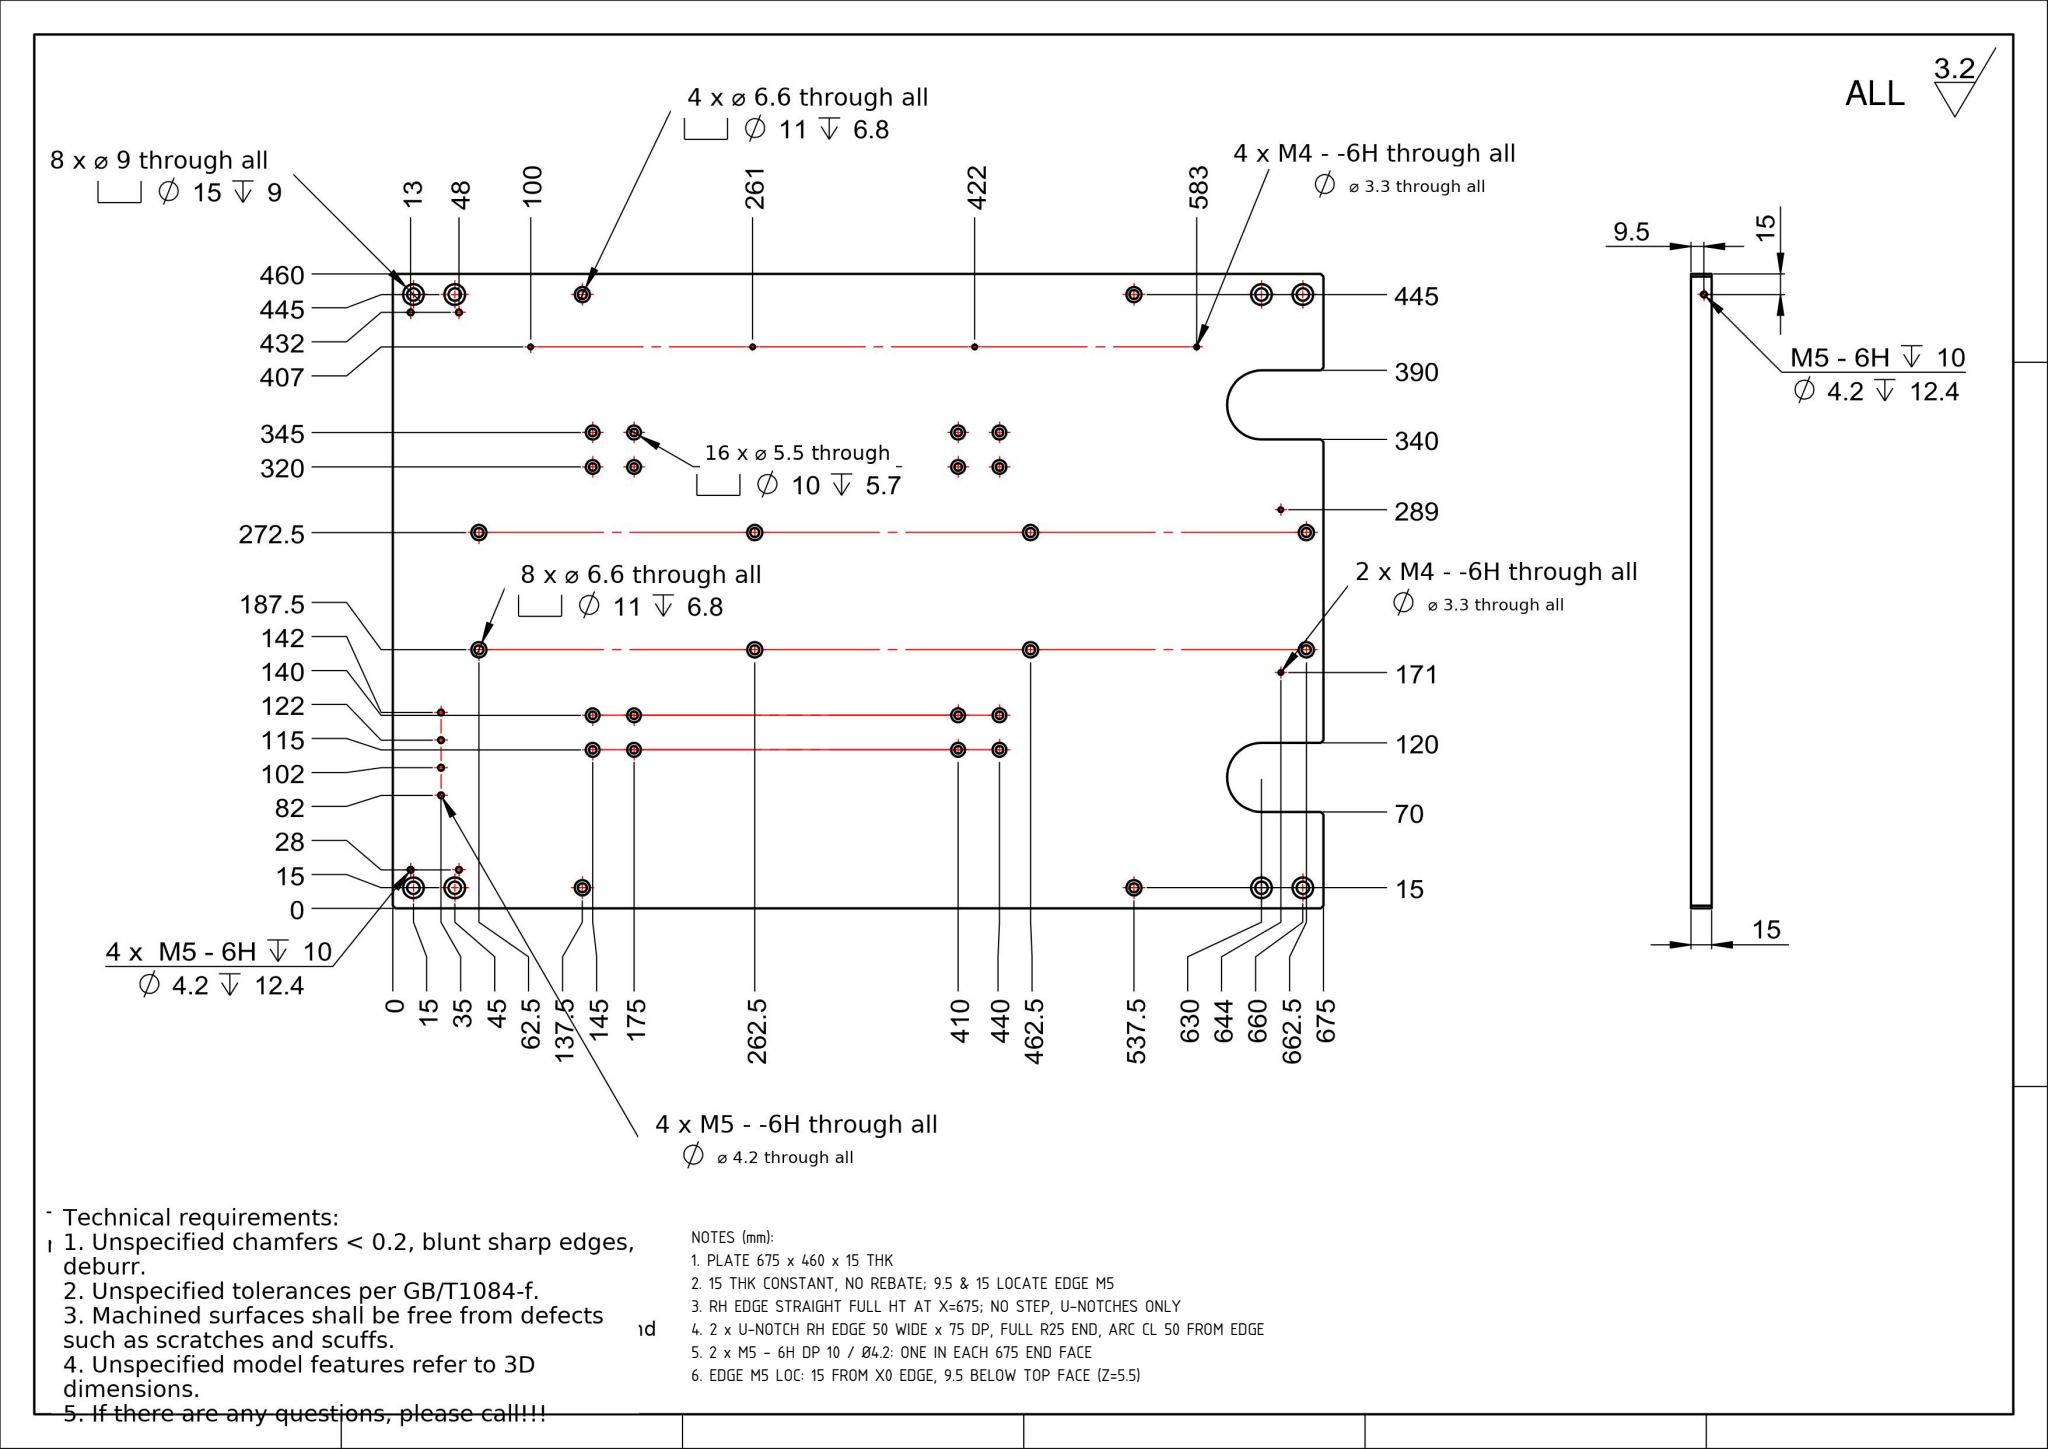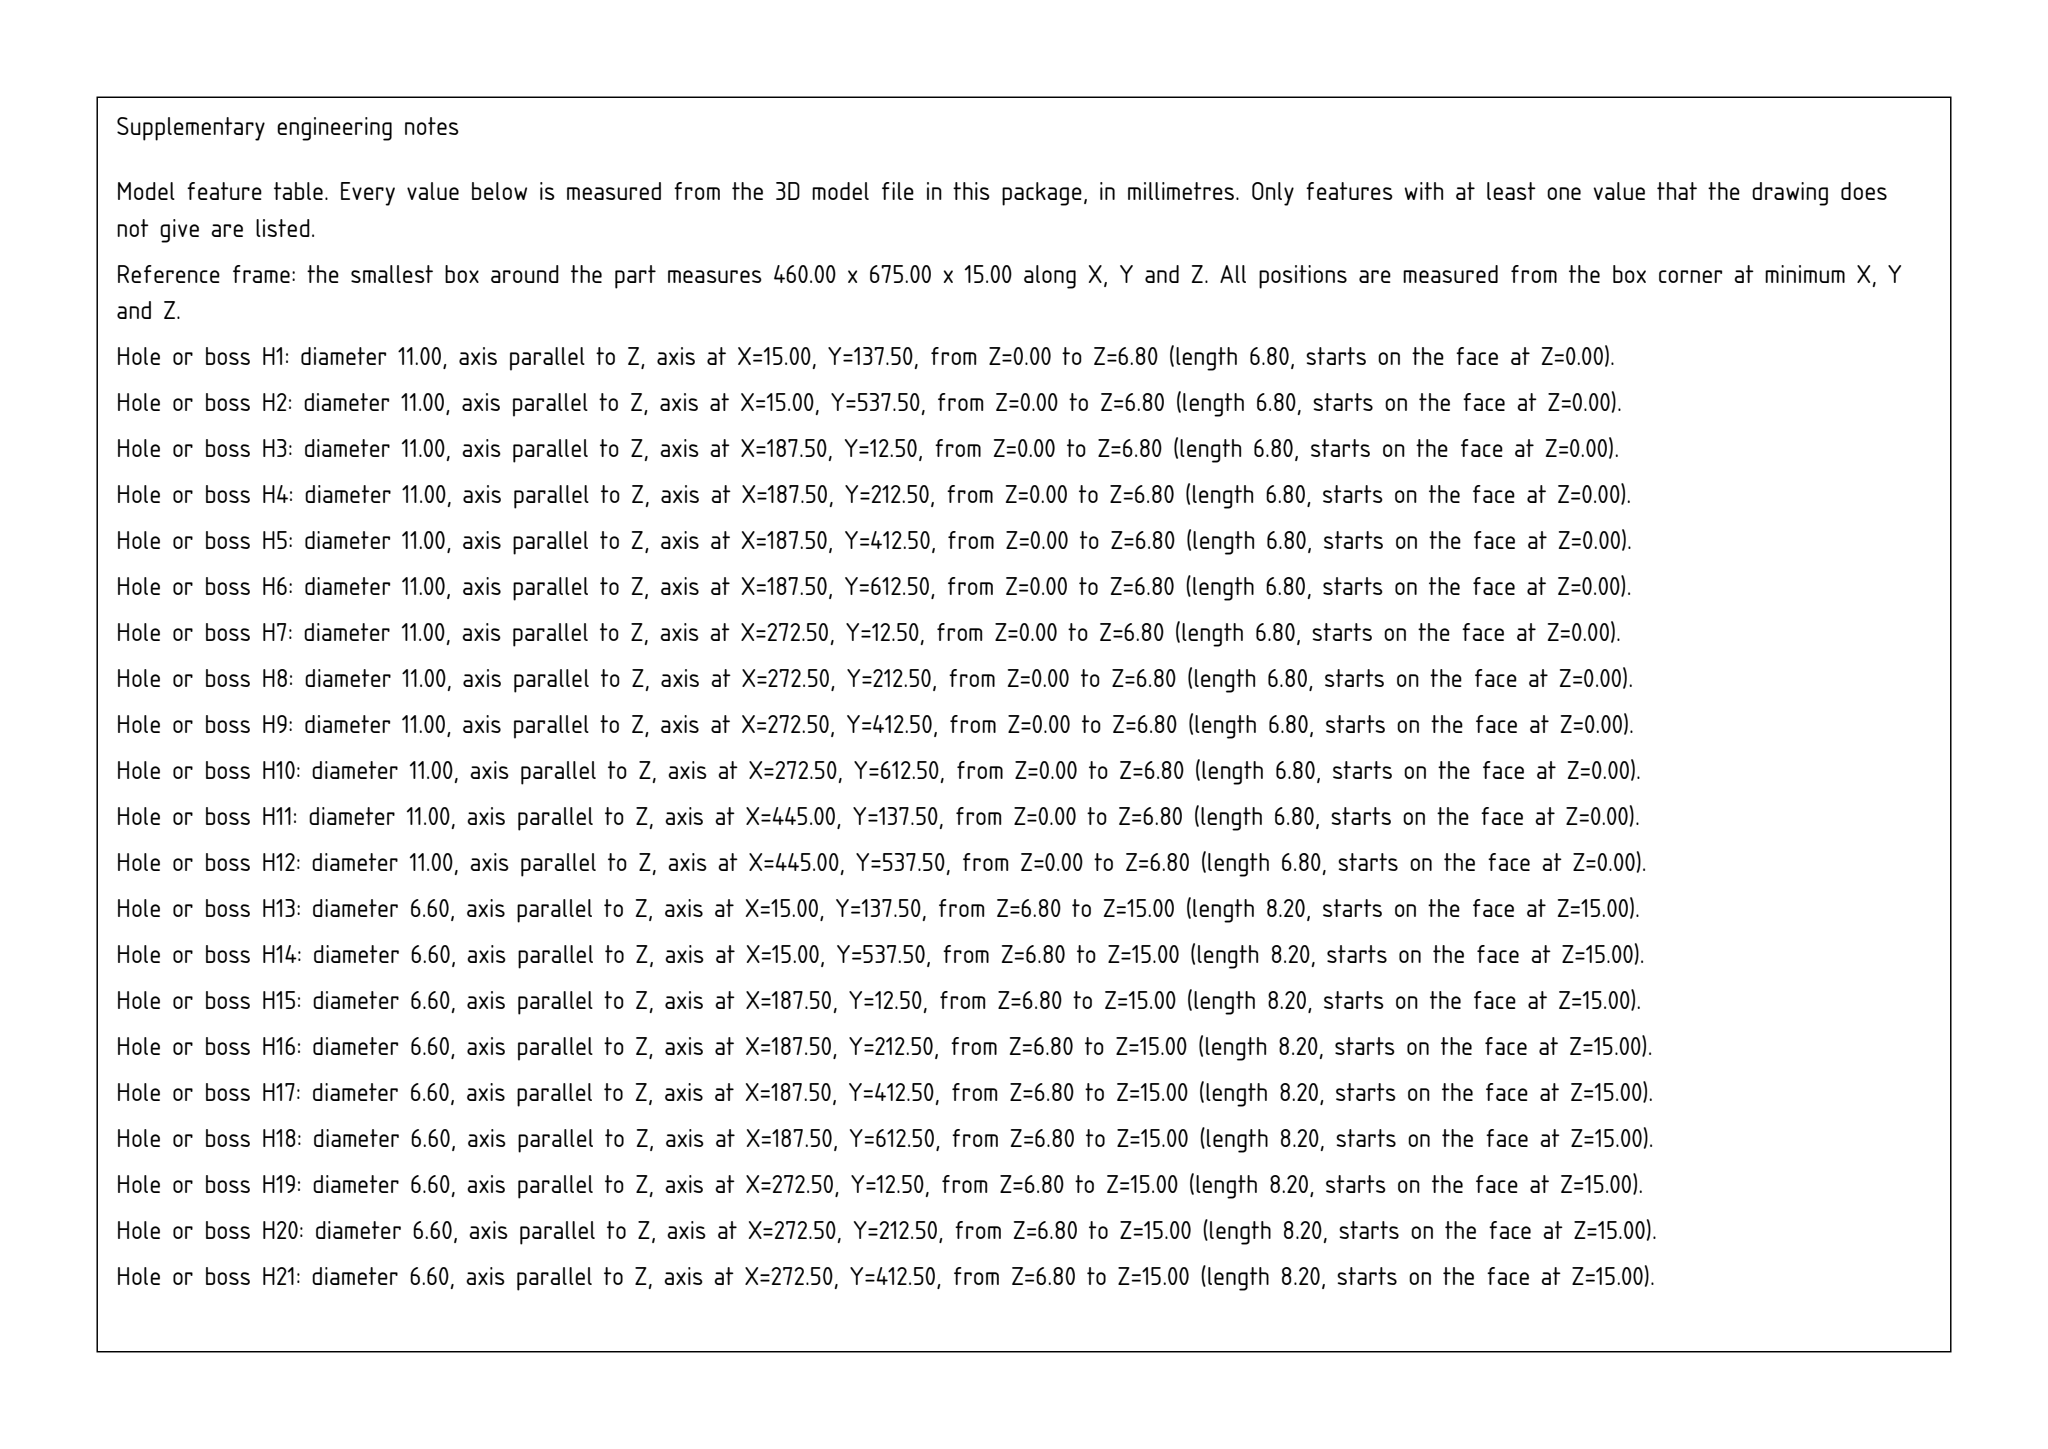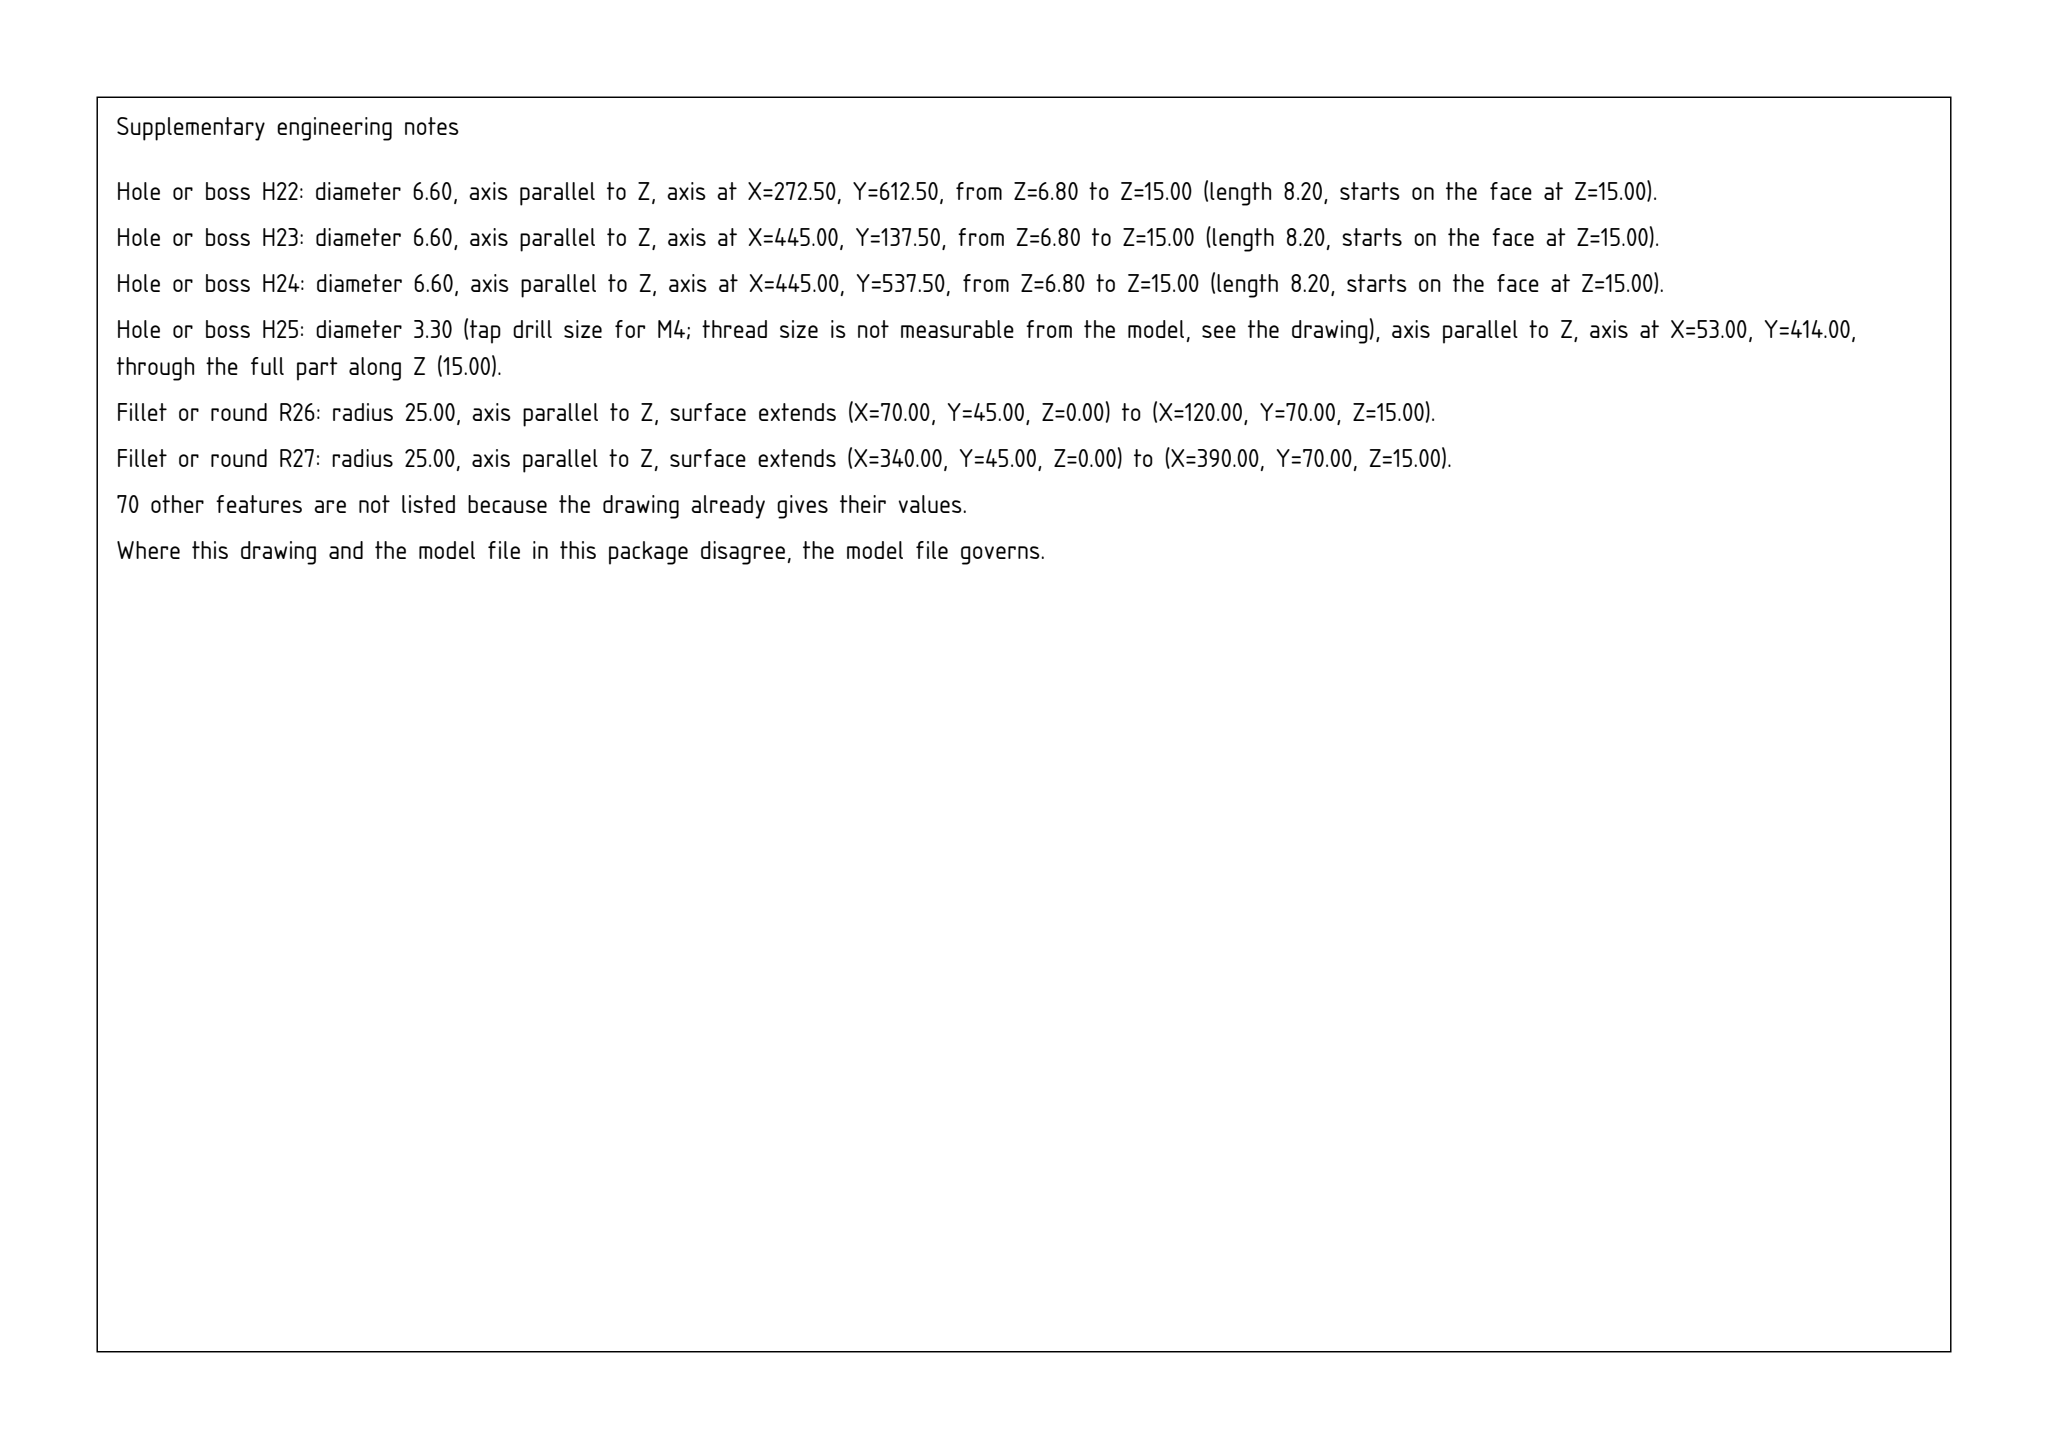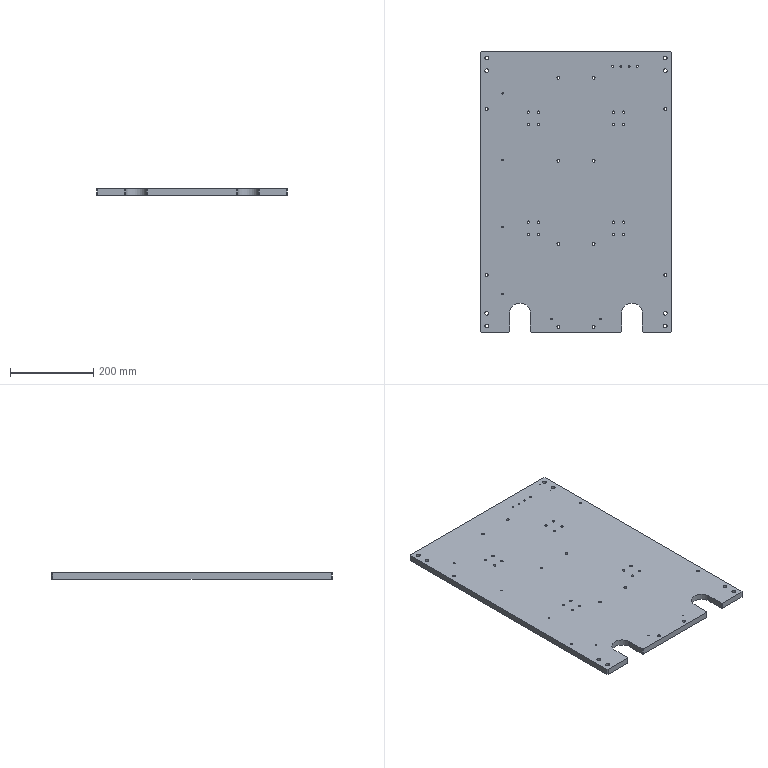Part | SolidWorks | mm | 1 solid | 240 faces | box 460 x 675 x 15 mm | volume 4520295 mm3 | cylinder 176 | plane 56 | cone 8 | commonest cylinder face diameters 10 x32 5.5 x32 11 x24 6.6 x24 4.2 x18 15 x16 9 x16 3.3 x12
Drawing notes:
PLATE 675 x 460 x 15 THK | from the solid: bbox_xyz [460,675,15]
15 THK CONSTANT, NO REBATE; 9.5 & 15 LOCATE EDGE M5 | from the solid: z-planes only 0.0 and 15.0 full faces = uniform plate; Ø4.2 y-axis hole at x=15, z=5.5 (9.5 below z=15 face)
RH EDGE STRAIGHT FULL HT AT X=675; NO STEP, U-NOTCHES ONLY | from the solid: axis_planes ['y',0.0] count 3 coplanar RH-edge faces (drawing X=675); only other y-plane is 675 (LH edge)
2 x U-NOTCH RH EDGE 50 WIDE x 75 DP, FULL R25 END, ARC CL 50 FROM EDGE | from the solid: notch flats x=70/120 and x=340/390 = 50 wide, running in from y=0 RH edge; full R25 end, arc centre 50 in = 75 total depth
2 x M5 - 6H DP 10 / Ø4.2: ONE IN EACH 675 END FACE | from the solid: cylinders [4.2,"y",[15.0,null,5.5],7.8, count 2] - axis along Y, one hole in each y-end face (y=0 and y=675) of 460x675x15 bbox
EDGE M5 LOC: 15 FROM X0 EDGE, 9.5 BELOW TOP FACE (Z=5.5) | from the solid: hole axis at x=15.0, z=5.5; thickness 15 so 15-5.5=9.5 from top face, matching 9.5 & 15 in side view
build123d program:
from build123d import *

# Parameters (mm, degrees)
SKETCH1_W                                         = 460
SKETCH1_H                                         = 675
BOSS_EXTRUDE1_DEPTH                               = 7.5
HOLE_SIZE_ACCORDING_TO_HEXAGON_SOCKET_D           = 6.6
HOLE_SIZE_ACCORDING_TO_HEXAGON_SOCKET_CBORE_D     = 11
HOLE_SIZE_ACCORDING_TO_HEXAGON_SOCKET_CBORE_DEPTH = 6.8
M8_HEX_SOCKET_HEAD_CAP_SCREW_CBORE3_D             = 9
M8_HEX_SOCKET_HEAD_CAP_SCREW_CBORE3_CBORE_D       = 15
M8_HEX_SOCKET_HEAD_CAP_SCREW_CBORE3_CBORE_DEPTH   = 9
M5_TAPPED_HOLE2_D                                 = 4.2
HOLE_SIZE_ACCORDING_TO_HEXAGON_SO_2_D             = 6.6
HOLE_SIZE_ACCORDING_TO_HEXAGON_SO_2_CBORE_D       = 11
HOLE_SIZE_ACCORDING_TO_HEXAGON_SO_2_CBORE_DEPTH   = 6.8
M4_TAPPED_HOLE3_D                                 = 3.3
LPATTERN3_COUNT                                   = 4
LPATTERN3_PITCH                                   = 161
HOLE_SIZE_ACCORDING_TO_HEXAGON_SO_3_D             = 5.5
HOLE_SIZE_ACCORDING_TO_HEXAGON_SO_3_CBORE_D       = 10
HOLE_SIZE_ACCORDING_TO_HEXAGON_SO_3_CBORE_DEPTH   = 5.7
LPATTERN4_COUNT                                   = 2
LPATTERN4_PITCH                                   = 265
MIRROR1_COPY_1_D                                  = 5.5
MIRROR1_COPY_1_CBORE_D                            = 10
MIRROR1_COPY_1_CBORE_DEPTH                        = 5.7
CHAMFER1_SIZE                                     = 2
M5_TAPPED_HOLE3_D                                 = 4.2
M5_TAPPED_HOLE3_DEPTH                             = 12.4
M5_TAPPED_HOLE3_TIP                               = 1.262
M4_TAPPED_HOLE4_D                                 = 3.3
HOLE_SIZE_ACCORDING_TO_HEXAGON_SO_4_D             = 6.6
HOLE_SIZE_ACCORDING_TO_HEXAGON_SO_4_CBORE_D       = 11
HOLE_SIZE_ACCORDING_TO_HEXAGON_SO_4_CBORE_DEPTH   = 6.8
LPATTERN8_COUNT                                   = 4
LPATTERN8_PITCH                                   = 200
M5_TAPPED_HOLE4_D                                 = 4.2
M5_TAPPED_HOLE4_DEPTH                             = 12.4
M5_TAPPED_HOLE4_TIP                               = 1.262
CUT_EXTRUDE1_DEPTH                                = 409.695
CHAMFER2_SIZE                                     = 2


with BuildPart() as part:
    # Sketch1 → Boss-Extrude1 (new, symmetric)
    with BuildSketch(Plane.XY):
        Rectangle(SKETCH1_W, SKETCH1_H)
    extrude(amount=BOSS_EXTRUDE1_DEPTH, both=True)

    # Hole Size _ according to_ Hexagon Socket (through all)
    with Locations(Plane(origin=(0, 0, -7.5), x_dir=(1, 0, 0), z_dir=(0, 0, -1))):
        with Locations((42.5, 325), (-42.5, 325)):
            CounterBoreHole(HOLE_SIZE_ACCORDING_TO_HEXAGON_SOCKET_D / 2, HOLE_SIZE_ACCORDING_TO_HEXAGON_SOCKET_CBORE_D / 2, HOLE_SIZE_ACCORDING_TO_HEXAGON_SOCKET_CBORE_DEPTH)

    # M8 Hex Socket Head Cap Screw CBORE3 (through all)
    with Locations(Plane(origin=(0, 0, -7.5), x_dir=(-1, 0, 0), z_dir=(0, 0, -1))):
        with Locations((-215, -322.5), (215, -322.5), (-215, -292.5), (215, -292.5), (215, 292.5), (215, 322.5), (-215, 322.5), (-215, 292.5)):
            CounterBoreHole(M8_HEX_SOCKET_HEAD_CAP_SCREW_CBORE3_D / 2, M8_HEX_SOCKET_HEAD_CAP_SCREW_CBORE3_CBORE_D / 2, M8_HEX_SOCKET_HEAD_CAP_SCREW_CBORE3_CBORE_DEPTH)

    # M5 Tapped Hole2 (through all)
    with Locations(Plane.XY.offset(7.5)):
        with Locations((88, 302.5), (108, 302.5), (128, 302.5), (148, 302.5)):
            Hole(M5_TAPPED_HOLE2_D / 2)

    # Hole Size _ according to_ Hexagon So 2 (through all)
    with Locations(Plane(origin=(0, 0, -7.5), x_dir=(-1, 0, 0), z_dir=(0, 0, -1))):
        with Locations((215, 200), (-215, 200), (215, -200), (-215, -200)):
            CounterBoreHole(HOLE_SIZE_ACCORDING_TO_HEXAGON_SO_2_D / 2, HOLE_SIZE_ACCORDING_TO_HEXAGON_SO_2_CBORE_D / 2, HOLE_SIZE_ACCORDING_TO_HEXAGON_SO_2_CBORE_DEPTH)

    # M4 Tapped Hole3 (through all)
    with Locations(Plane.XY.offset(7.5)):
        with Locations((-177, 237.5)):
            m4_tapped_hole3 = Hole(M4_TAPPED_HOLE3_D / 2)

    # LPattern3: M4 Tapped Hole3 ×4
    with Locations(*[(0, -i * LPATTERN3_PITCH, 0) for i in range(1, LPATTERN3_COUNT)]):
        add(m4_tapped_hole3, mode=Mode.SUBTRACT)

    # Hole Size _ according to_ Hexagon So 3 (through all)
    with Locations(Plane(origin=(0, 0, -7.5), x_dir=(1, 0, 0), z_dir=(0, 0, -1))):
        with Locations((90, -192.5), (90, -162.5), (115, -192.5), (115, -162.5)):
            hole_size_according_to_hexagon_so_3 = CounterBoreHole(HOLE_SIZE_ACCORDING_TO_HEXAGON_SO_3_D / 2, HOLE_SIZE_ACCORDING_TO_HEXAGON_SO_3_CBORE_D / 2, HOLE_SIZE_ACCORDING_TO_HEXAGON_SO_3_CBORE_DEPTH)

    # LPattern4: Hole Size _ according to_ Hexagon So 3 ×2
    with Locations(*[(0, -i * LPATTERN4_PITCH, 0) for i in range(1, LPATTERN4_COUNT)]):
        add(hole_size_according_to_hexagon_so_3, mode=Mode.SUBTRACT)

    # Mirror1: Hole Size _ according to_ Hexagon So 3 across plane
    add(hole_size_according_to_hexagon_so_3.mirror(Plane(origin=(0, 0, 0), x_dir=(0, 0, 1), z_dir=(1, 0, 0))), mode=Mode.SUBTRACT)

    # Mirror1 copy 1 (through all)
    with Locations(Plane(origin=(0, -265, -7.5), x_dir=(-1, 0, 0), z_dir=(0, 0, -1))):
        with Locations((90, 192.5), (90, 162.5), (115, 192.5), (115, 162.5)):
            CounterBoreHole(MIRROR1_COPY_1_D / 2, MIRROR1_COPY_1_CBORE_D / 2, MIRROR1_COPY_1_CBORE_DEPTH)

    # Chamfer1
    chamfer1_edges = [part.edges().sort_by_distance(p)[0] for p in [
        (230, -337.5, 0),
        (-230, -337.5, 0),
        (-230, 337.5, 0),
        (230, 337.5, 0),
    ]]
    chamfer(chamfer1_edges, length=CHAMFER1_SIZE)

    # M5 Tapped Hole3
    with Locations(Plane(origin=(0, 0, -7.5), x_dir=(-1, 0, 0), z_dir=(0, 0, -1))):
        with Locations((202, 324.5), (202, 289.5), (-202, 289.5), (-202, 324.5)):
            Hole(M5_TAPPED_HOLE3_D / 2, depth=M5_TAPPED_HOLE3_DEPTH)
            with Locations((0, 0, -(M5_TAPPED_HOLE3_DEPTH + M5_TAPPED_HOLE3_TIP / 2))):  # 118° drill point
                Cone(0, M5_TAPPED_HOLE3_D / 2, M5_TAPPED_HOLE3_TIP, mode=Mode.SUBTRACT)

    # M4 Tapped Hole4 (through all)
    with Locations(Plane(origin=(0, 0, -7.5), x_dir=(-1, 0, 0), z_dir=(0, 0, -1))):
        with Locations((-59, -306.5), (59, -306.5)):
            Hole(M4_TAPPED_HOLE4_D / 2)

    # Hole Size _ according to_ Hexagon So 4 (through all)
    with Locations(Plane(origin=(0, 0, -7.5), x_dir=(-1, 0, 0), z_dir=(0, 0, -1))):
        with Locations((-42.5, -325), (42.5, -325)):
            hole_size_according_to_hexagon_so_4 = CounterBoreHole(HOLE_SIZE_ACCORDING_TO_HEXAGON_SO_4_D / 2, HOLE_SIZE_ACCORDING_TO_HEXAGON_SO_4_CBORE_D / 2, HOLE_SIZE_ACCORDING_TO_HEXAGON_SO_4_CBORE_DEPTH)

    # LPattern8: Hole Size _ according to_ Hexagon So 4 ×4
    with Locations(*[(0, i * LPATTERN8_PITCH, 0) for i in range(1, LPATTERN8_COUNT)]):
        add(hole_size_according_to_hexagon_so_4, mode=Mode.SUBTRACT)

    # M5 Tapped Hole4
    with Locations(Plane(origin=(0, 337.5, 0), x_dir=(1, 0, 0), z_dir=(0, 1, 0))):
        with Locations((-215, 2)):
            Hole(M5_TAPPED_HOLE4_D / 2, depth=M5_TAPPED_HOLE4_DEPTH)
            with Locations((0, 0, -(M5_TAPPED_HOLE4_DEPTH + M5_TAPPED_HOLE4_TIP / 2))):  # 118° drill point
                Cone(0, M5_TAPPED_HOLE4_D / 2, M5_TAPPED_HOLE4_TIP, mode=Mode.SUBTRACT)

    # Sketch40 → Cut-Extrude1 (cut, through all)
    with BuildSketch(Plane(origin=(0, 0, -7.5), x_dir=(-1, 0, 0), z_dir=(0, 0, -1))):
        with BuildLine():
            Line((110, -382.5), (110, -292.5))
            ThreePointArc((110, -292.5), (135, -267.5), (160, -292.5))
            Line((160, -292.5), (160, -382.5))
            ThreePointArc((160, -382.5), (135, -407.5), (110, -382.5))
        make_face()
        with BuildLine():
            Line((-110, -382.5), (-110, -292.5))
            ThreePointArc((-110, -292.5), (-135, -267.5), (-160, -292.5))
            Line((-160, -292.5), (-160, -382.5))
            ThreePointArc((-160, -382.5), (-135, -407.5), (-110, -382.5))
        make_face()
    extrude(amount=-CUT_EXTRUDE1_DEPTH, mode=Mode.SUBTRACT)

    # Chamfer2
    chamfer2_edges = [part.edges().sort_by_distance(p)[0] for p in [
        (-160, -337.5, 0),
        (-110, -337.5, 0),
        (160, -337.5, 0),
        (110, -337.5, 0),
    ]]
    chamfer(chamfer2_edges, length=CHAMFER2_SIZE)


solid = part.part